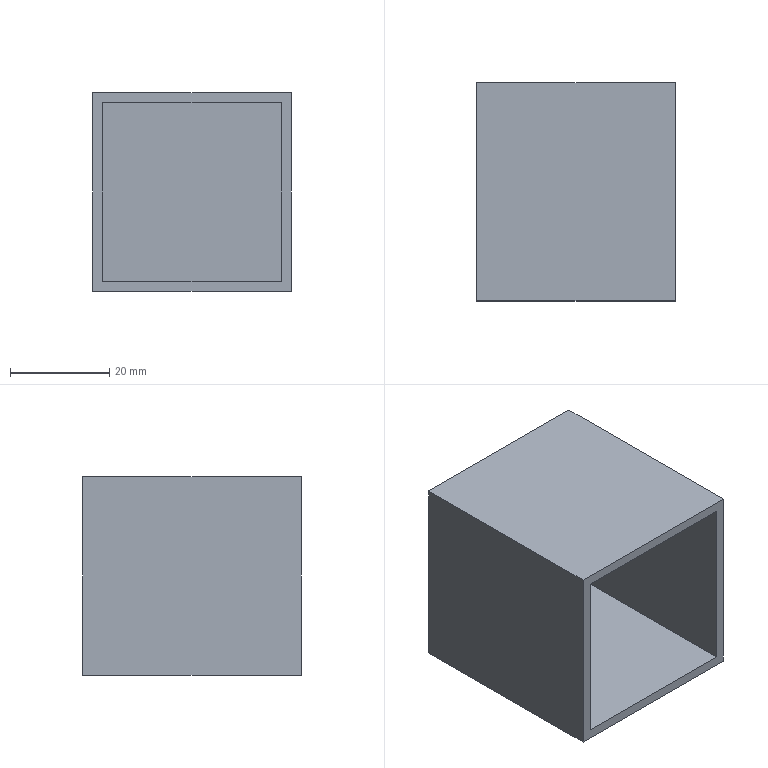Component | SolidWorks | Explosion-proofCasing-1 | 1 solid | 11 faces | box 40 x 44 x 40 mm | volume 15968 mm3 | plane 11 | material 45
build123d program:
from build123d import *

# Parameters (mm, degrees)
SKETCH1_W           = 40
SKETCH1_H           = 40
SKETCH1_W_2         = 36
SKETCH1_H_2         = 36
EXTRUDE_THIN1_DEPTH = 42
SKETCH2_W           = 40
SKETCH2_H           = 40
BOSS_EXTRUDE1_DEPTH = 2


with BuildPart() as part:
    # Sketch1 → Extrude-Thin1 (new body)
    with BuildSketch(Plane.XY):
        Rectangle(SKETCH1_W, SKETCH1_H)
        Rectangle(SKETCH1_W_2, SKETCH1_H_2, mode=Mode.SUBTRACT)
    extrude(amount=EXTRUDE_THIN1_DEPTH)

    # Sketch2 → Boss-Extrude1 (add)
    with BuildSketch(Plane(origin=(0, 0, 0), x_dir=(-1, 0, 0), z_dir=(0, 0, -1))):
        Rectangle(SKETCH2_W, SKETCH2_H)
    extrude(amount=BOSS_EXTRUDE1_DEPTH)


solid = part.part

# Placed as in the assembly
solid = solid.moved(Location((-371.359, -405.185, 1062), (90, 0, 0)))
STEP:
#1=COLOUR_RGB('',0.7922,0.8196,0.9333);
#2=FILL_AREA_STYLE_COLOUR('',#1);
#3=FILL_AREA_STYLE('',(#2));
#4=SURFACE_STYLE_FILL_AREA(#3);
#5=SURFACE_SIDE_STYLE('',(#4));
#6=SURFACE_STYLE_USAGE(.BOTH.,#5);
#7=PRESENTATION_STYLE_ASSIGNMENT((#6));
#8=CARTESIAN_POINT('',(-15.408,-17.606,42.598));
#9=VERTEX_POINT('',#8);
#10=CARTESIAN_POINT('',(-15.408,-17.606,41.024));
#11=VERTEX_POINT('',#10);
#12=CARTESIAN_POINT('',(-15.408,-17.606,41.024));
#13=DIRECTION('',(-0.,0.,-1.));
#14=VECTOR('',#13,39.37);
#15=LINE('',#12,#14);
#16=EDGE_CURVE('',#9,#11,#15,.T.);
#17=ORIENTED_EDGE('',*,*,#16,.T.);
#18=CARTESIAN_POINT('',(-13.833,-17.606,41.024));
#19=VERTEX_POINT('',#18);
#20=CARTESIAN_POINT('',(-13.833,-17.606,41.024));
#21=DIRECTION('',(1.,0.,0.));
#22=VECTOR('',#21,39.37);
#23=LINE('',#20,#22);
#24=EDGE_CURVE('',#11,#19,#23,.T.);
#25=ORIENTED_EDGE('',*,*,#24,.T.);
#26=CARTESIAN_POINT('',(-13.833,-17.606,42.598));
#27=VERTEX_POINT('',#26);
#28=CARTESIAN_POINT('',(-13.833,-17.606,41.024));
#29=DIRECTION('',(0.,0.,1.));
#30=VECTOR('',#29,39.37);
#31=LINE('',#28,#30);
#32=EDGE_CURVE('',#19,#27,#31,.T.);
#33=ORIENTED_EDGE('',*,*,#32,.T.);
#34=CARTESIAN_POINT('',(-13.833,-17.606,42.598));
#35=DIRECTION('',(-1.,0.,-0.));
#36=VECTOR('',#35,39.37);
#37=LINE('',#34,#36);
#38=EDGE_CURVE('',#27,#9,#37,.T.);
#39=ORIENTED_EDGE('',*,*,#38,.T.);
#40=EDGE_LOOP('',(#17,#25,#33,#39));
#41=FACE_OUTER_BOUND('',#40,.T.);
#42=CARTESIAN_POINT('',(-15.329,-17.606,41.102));
#43=VERTEX_POINT('',#42);
#44=CARTESIAN_POINT('',(-13.912,-17.606,41.102));
#45=VERTEX_POINT('',#44);
#46=CARTESIAN_POINT('',(-13.833,-17.606,41.102));
#47=DIRECTION('',(1.,0.,0.));
#48=VECTOR('',#47,39.37);
#49=LINE('',#46,#48);
#50=EDGE_CURVE('',#43,#45,#49,.T.);
#51=ORIENTED_EDGE('',*,*,#50,.F.);
#52=CARTESIAN_POINT('',(-15.329,-17.606,42.52));
#53=VERTEX_POINT('',#52);
#54=CARTESIAN_POINT('',(-15.329,-17.606,41.024));
#55=DIRECTION('',(-0.,0.,-1.));
#56=VECTOR('',#55,39.37);
#57=LINE('',#54,#56);
#58=EDGE_CURVE('',#53,#43,#57,.T.);
#59=ORIENTED_EDGE('',*,*,#58,.F.);
#60=CARTESIAN_POINT('',(-13.912,-17.606,42.52));
#61=VERTEX_POINT('',#60);
#62=CARTESIAN_POINT('',(-13.833,-17.606,42.52));
#63=DIRECTION('',(-1.,0.,-0.));
#64=VECTOR('',#63,39.37);
#65=LINE('',#62,#64);
#66=EDGE_CURVE('',#61,#53,#65,.T.);
#67=ORIENTED_EDGE('',*,*,#66,.F.);
#68=CARTESIAN_POINT('',(-13.912,-17.606,41.024));
#69=DIRECTION('',(0.,0.,1.));
#70=VECTOR('',#69,39.37);
#71=LINE('',#68,#70);
#72=EDGE_CURVE('',#45,#61,#71,.T.);
#73=ORIENTED_EDGE('',*,*,#72,.F.);
#74=EDGE_LOOP('',(#51,#59,#67,#73));
#75=FACE_BOUND('',#74,.T.);
#76=CARTESIAN_POINT('',(-14.62,-17.606,41.811));
#77=DIRECTION('',(0.,-1.,0.));
#78=DIRECTION('',(1.,0.,0.));
#79=AXIS2_PLACEMENT_3D('',#76,#77,#78);
#80=PLANE('',#79);
#81=ADVANCED_FACE('',(#41,#75),#80,.T.);
#82=CARTESIAN_POINT('',(-15.408,-15.873,42.598));
#83=VERTEX_POINT('',#82);
#84=CARTESIAN_POINT('',(-15.408,-17.606,42.598));
#85=DIRECTION('',(0.,1.,0.));
#86=VECTOR('',#85,39.37);
#87=LINE('',#84,#86);
#88=EDGE_CURVE('',#9,#83,#87,.T.);
#89=ORIENTED_EDGE('',*,*,#88,.T.);
#90=CARTESIAN_POINT('',(-15.408,-15.873,41.024));
#91=VERTEX_POINT('',#90);
#92=CARTESIAN_POINT('',(-15.408,-15.873,41.024));
#93=DIRECTION('',(0.,0.,1.));
#94=VECTOR('',#93,39.37);
#95=LINE('',#92,#94);
#96=EDGE_CURVE('',#91,#83,#95,.T.);
#97=ORIENTED_EDGE('',*,*,#96,.F.);
#98=CARTESIAN_POINT('',(-15.408,-17.606,41.024));
#99=DIRECTION('',(0.,1.,0.));
#100=VECTOR('',#99,39.37);
#101=LINE('',#98,#100);
#102=EDGE_CURVE('',#11,#91,#101,.T.);
#103=ORIENTED_EDGE('',*,*,#102,.F.);
#104=ORIENTED_EDGE('',*,*,#16,.F.);
#105=EDGE_LOOP('',(#89,#97,#103,#104));
#106=FACE_OUTER_BOUND('',#105,.T.);
#107=CARTESIAN_POINT('',(-15.408,-17.606,41.024));
#108=DIRECTION('',(1.,0.,-0.));
#109=DIRECTION('',(0.,0.,1.));
#110=AXIS2_PLACEMENT_3D('',#107,#108,#109);
#111=PLANE('',#110);
#112=ADVANCED_FACE('',(#106),#111,.F.);
#113=ORIENTED_EDGE('',*,*,#102,.T.);
#114=CARTESIAN_POINT('',(-13.833,-15.873,41.024));
#115=VERTEX_POINT('',#114);
#116=CARTESIAN_POINT('',(-13.833,-15.873,41.024));
#117=DIRECTION('',(-1.,0.,-0.));
#118=VECTOR('',#117,39.37);
#119=LINE('',#116,#118);
#120=EDGE_CURVE('',#115,#91,#119,.T.);
#121=ORIENTED_EDGE('',*,*,#120,.F.);
#122=CARTESIAN_POINT('',(-13.833,-17.606,41.024));
#123=DIRECTION('',(0.,1.,0.));
#124=VECTOR('',#123,39.37);
#125=LINE('',#122,#124);
#126=EDGE_CURVE('',#19,#115,#125,.T.);
#127=ORIENTED_EDGE('',*,*,#126,.F.);
#128=ORIENTED_EDGE('',*,*,#24,.F.);
#129=EDGE_LOOP('',(#113,#121,#127,#128));
#130=FACE_OUTER_BOUND('',#129,.T.);
#131=CARTESIAN_POINT('',(-13.833,-17.606,41.024));
#132=DIRECTION('',(-0.,0.,1.));
#133=DIRECTION('',(-1.,0.,-0.));
#134=AXIS2_PLACEMENT_3D('',#131,#132,#133);
#135=PLANE('',#134);
#136=ADVANCED_FACE('',(#130),#135,.F.);
#137=ORIENTED_EDGE('',*,*,#126,.T.);
#138=CARTESIAN_POINT('',(-13.833,-15.873,42.598));
#139=VERTEX_POINT('',#138);
#140=CARTESIAN_POINT('',(-13.833,-15.873,42.598));
#141=DIRECTION('',(0.,0.,-1.));
#142=VECTOR('',#141,39.37);
#143=LINE('',#140,#142);
#144=EDGE_CURVE('',#139,#115,#143,.T.);
#145=ORIENTED_EDGE('',*,*,#144,.F.);
#146=CARTESIAN_POINT('',(-13.833,-17.606,42.598));
#147=DIRECTION('',(0.,1.,0.));
#148=VECTOR('',#147,39.37);
#149=LINE('',#146,#148);
#150=EDGE_CURVE('',#27,#139,#149,.T.);
#151=ORIENTED_EDGE('',*,*,#150,.F.);
#152=ORIENTED_EDGE('',*,*,#32,.F.);
#153=EDGE_LOOP('',(#137,#145,#151,#152));
#154=FACE_OUTER_BOUND('',#153,.T.);
#155=CARTESIAN_POINT('',(-13.833,-17.606,41.024));
#156=DIRECTION('',(-1.,0.,0.));
#157=DIRECTION('',(0.,-1.,0.));
#158=AXIS2_PLACEMENT_3D('',#155,#156,#157);
#159=PLANE('',#158);
#160=ADVANCED_FACE('',(#154),#159,.F.);
#161=ORIENTED_EDGE('',*,*,#150,.T.);
#162=CARTESIAN_POINT('',(-15.408,-15.873,42.598));
#163=DIRECTION('',(1.,0.,0.));
#164=VECTOR('',#163,39.37);
#165=LINE('',#162,#164);
#166=EDGE_CURVE('',#83,#139,#165,.T.);
#167=ORIENTED_EDGE('',*,*,#166,.F.);
#168=ORIENTED_EDGE('',*,*,#88,.F.);
#169=ORIENTED_EDGE('',*,*,#38,.F.);
#170=EDGE_LOOP('',(#161,#167,#168,#169));
#171=FACE_OUTER_BOUND('',#170,.T.);
#172=CARTESIAN_POINT('',(-13.833,-17.606,42.598));
#173=DIRECTION('',(0.,0.,-1.));
#174=DIRECTION('',(1.,0.,0.));
#175=AXIS2_PLACEMENT_3D('',#172,#173,#174);
#176=PLANE('',#175);
#177=ADVANCED_FACE('',(#171),#176,.F.);
#178=CARTESIAN_POINT('',(-15.329,-15.952,42.52));
#179=VERTEX_POINT('',#178);
#180=CARTESIAN_POINT('',(-15.329,-15.952,41.102));
#181=VERTEX_POINT('',#180);
#182=CARTESIAN_POINT('',(-15.329,-15.952,41.024));
#183=DIRECTION('',(-0.,0.,-1.));
#184=VECTOR('',#183,39.37);
#185=LINE('',#182,#184);
#186=EDGE_CURVE('',#179,#181,#185,.T.);
#187=ORIENTED_EDGE('',*,*,#186,.F.);
#188=CARTESIAN_POINT('',(-15.329,-17.606,42.52));
#189=DIRECTION('',(0.,1.,0.));
#190=VECTOR('',#189,39.37);
#191=LINE('',#188,#190);
#192=EDGE_CURVE('',#53,#179,#191,.T.);
#193=ORIENTED_EDGE('',*,*,#192,.F.);
#194=ORIENTED_EDGE('',*,*,#58,.T.);
#195=CARTESIAN_POINT('',(-15.329,-17.606,41.102));
#196=DIRECTION('',(0.,1.,0.));
#197=VECTOR('',#196,39.37);
#198=LINE('',#195,#197);
#199=EDGE_CURVE('',#43,#181,#198,.T.);
#200=ORIENTED_EDGE('',*,*,#199,.T.);
#201=EDGE_LOOP('',(#187,#193,#194,#200));
#202=FACE_OUTER_BOUND('',#201,.T.);
#203=CARTESIAN_POINT('',(-15.329,-17.606,41.024));
#204=DIRECTION('',(1.,0.,-0.));
#205=DIRECTION('',(0.,0.,1.));
#206=AXIS2_PLACEMENT_3D('',#203,#204,#205);
#207=PLANE('',#206);
#208=ADVANCED_FACE('',(#202),#207,.T.);
#209=CARTESIAN_POINT('',(-13.912,-15.952,41.102));
#210=VERTEX_POINT('',#209);
#211=CARTESIAN_POINT('',(-13.833,-15.952,41.102));
#212=DIRECTION('',(1.,0.,0.));
#213=VECTOR('',#212,39.37);
#214=LINE('',#211,#213);
#215=EDGE_CURVE('',#181,#210,#214,.T.);
#216=ORIENTED_EDGE('',*,*,#215,.F.);
#217=ORIENTED_EDGE('',*,*,#199,.F.);
#218=ORIENTED_EDGE('',*,*,#50,.T.);
#219=CARTESIAN_POINT('',(-13.912,-17.606,41.102));
#220=DIRECTION('',(0.,1.,0.));
#221=VECTOR('',#220,39.37);
#222=LINE('',#219,#221);
#223=EDGE_CURVE('',#45,#210,#222,.T.);
#224=ORIENTED_EDGE('',*,*,#223,.T.);
#225=EDGE_LOOP('',(#216,#217,#218,#224));
#226=FACE_OUTER_BOUND('',#225,.T.);
#227=CARTESIAN_POINT('',(-13.833,-17.606,41.102));
#228=DIRECTION('',(-0.,0.,1.));
#229=DIRECTION('',(-1.,0.,-0.));
#230=AXIS2_PLACEMENT_3D('',#227,#228,#229);
#231=PLANE('',#230);
#232=ADVANCED_FACE('',(#226),#231,.T.);
#233=CARTESIAN_POINT('',(-13.912,-15.952,42.52));
#234=VERTEX_POINT('',#233);
#235=CARTESIAN_POINT('',(-13.912,-15.952,41.024));
#236=DIRECTION('',(0.,0.,1.));
#237=VECTOR('',#236,39.37);
#238=LINE('',#235,#237);
#239=EDGE_CURVE('',#210,#234,#238,.T.);
#240=ORIENTED_EDGE('',*,*,#239,.F.);
#241=ORIENTED_EDGE('',*,*,#223,.F.);
#242=ORIENTED_EDGE('',*,*,#72,.T.);
#243=CARTESIAN_POINT('',(-13.912,-17.606,42.52));
#244=DIRECTION('',(0.,1.,0.));
#245=VECTOR('',#244,39.37);
#246=LINE('',#243,#245);
#247=EDGE_CURVE('',#61,#234,#246,.T.);
#248=ORIENTED_EDGE('',*,*,#247,.T.);
#249=EDGE_LOOP('',(#240,#241,#242,#248));
#250=FACE_OUTER_BOUND('',#249,.T.);
#251=CARTESIAN_POINT('',(-13.912,-17.606,41.024));
#252=DIRECTION('',(-1.,0.,0.));
#253=DIRECTION('',(0.,-1.,0.));
#254=AXIS2_PLACEMENT_3D('',#251,#252,#253);
#255=PLANE('',#254);
#256=ADVANCED_FACE('',(#250),#255,.T.);
#257=CARTESIAN_POINT('',(-13.833,-15.952,42.52));
#258=DIRECTION('',(-1.,0.,-0.));
#259=VECTOR('',#258,39.37);
#260=LINE('',#257,#259);
#261=EDGE_CURVE('',#234,#179,#260,.T.);
#262=ORIENTED_EDGE('',*,*,#261,.F.);
#263=ORIENTED_EDGE('',*,*,#247,.F.);
#264=ORIENTED_EDGE('',*,*,#66,.T.);
#265=ORIENTED_EDGE('',*,*,#192,.T.);
#266=EDGE_LOOP('',(#262,#263,#264,#265));
#267=FACE_OUTER_BOUND('',#266,.T.);
#268=CARTESIAN_POINT('',(-13.833,-17.606,42.52));
#269=DIRECTION('',(0.,0.,-1.));
#270=DIRECTION('',(1.,0.,0.));
#271=AXIS2_PLACEMENT_3D('',#268,#269,#270);
#272=PLANE('',#271);
#273=ADVANCED_FACE('',(#267),#272,.T.);
#274=ORIENTED_EDGE('',*,*,#261,.T.);
#275=ORIENTED_EDGE('',*,*,#186,.T.);
#276=ORIENTED_EDGE('',*,*,#215,.T.);
#277=ORIENTED_EDGE('',*,*,#239,.T.);
#278=EDGE_LOOP('',(#274,#275,#276,#277));
#279=FACE_OUTER_BOUND('',#278,.T.);
#280=CARTESIAN_POINT('',(-14.62,-15.952,41.811));
#281=DIRECTION('',(0.,1.,0.));
#282=DIRECTION('',(-1.,0.,0.));
#283=AXIS2_PLACEMENT_3D('',#280,#281,#282);
#284=PLANE('',#283);
#285=ADVANCED_FACE('',(#279),#284,.F.);
#286=ORIENTED_EDGE('',*,*,#120,.T.);
#287=ORIENTED_EDGE('',*,*,#96,.T.);
#288=ORIENTED_EDGE('',*,*,#166,.T.);
#289=ORIENTED_EDGE('',*,*,#144,.T.);
#290=EDGE_LOOP('',(#286,#287,#288,#289));
#291=FACE_OUTER_BOUND('',#290,.T.);
#292=CARTESIAN_POINT('',(-14.62,-15.873,41.811));
#293=DIRECTION('',(0.,1.,0.));
#294=DIRECTION('',(-1.,0.,0.));
#295=AXIS2_PLACEMENT_3D('',#292,#293,#294);
#296=PLANE('',#295);
#297=ADVANCED_FACE('',(#291),#296,.T.);
#298=CLOSED_SHELL('',(#81,#112,#136,#160,#177,#208,#232,#256,#273,#285,#297));
#299=MANIFOLD_SOLID_BREP('',#298);
#300=STYLED_ITEM('',(#7),#299);
#301=PRESENTATION_LAYER_ASSIGNMENT('','',(#300));
#302=CARTESIAN_POINT('',(0.,0.,0.));
#303=DIRECTION('',(0.,0.,1.));
#304=DIRECTION('',(1.,0.,0.));
#305=AXIS2_PLACEMENT_3D('',#302,#303,#304);
#306=(LENGTH_UNIT()NAMED_UNIT(*)SI_UNIT($,.METRE.));
#307=LENGTH_MEASURE_WITH_UNIT(LENGTH_MEASURE(0.0254),#306);
#308=DIMENSIONAL_EXPONENTS(1.,0.,0.,0.,0.,0.,0.);
#309=(CONVERSION_BASED_UNIT('',#307)LENGTH_UNIT()NAMED_UNIT(#308));
#310=UNCERTAINTY_MEASURE_WITH_UNIT(LENGTH_MEASURE(0.00001),#309,'','');
#311=(NAMED_UNIT(*)PLANE_ANGLE_UNIT()SI_UNIT($,.RADIAN.));
#312=(NAMED_UNIT(*)SI_UNIT($,.STERADIAN.)SOLID_ANGLE_UNIT());
#313=(GEOMETRIC_REPRESENTATION_CONTEXT(3)GLOBAL_UNCERTAINTY_ASSIGNED_CONTEXT((#310))GLOBAL_UNIT_ASSIGNED_CONTEXT((#309,#311,#312))REPRESENTATION_CONTEXT('',''));
#314=ADVANCED_BREP_SHAPE_REPRESENTATION('',(#299,#305),#313);
#315=(LENGTH_UNIT()NAMED_UNIT(*)SI_UNIT($,.METRE.));
#316=LENGTH_MEASURE_WITH_UNIT(LENGTH_MEASURE(0.0254),#315);
#317=DIMENSIONAL_EXPONENTS(1.,0.,0.,0.,0.,0.,0.);
#318=(CONVERSION_BASED_UNIT('',#316)LENGTH_UNIT()NAMED_UNIT(#317));
#319=UNCERTAINTY_MEASURE_WITH_UNIT(LENGTH_MEASURE(0.00001),#318,'','');
#320=(NAMED_UNIT(*)PLANE_ANGLE_UNIT()SI_UNIT($,.RADIAN.));
#321=(NAMED_UNIT(*)SI_UNIT($,.STERADIAN.)SOLID_ANGLE_UNIT());
#322=(GEOMETRIC_REPRESENTATION_CONTEXT(3)GLOBAL_UNCERTAINTY_ASSIGNED_CONTEXT((#319))GLOBAL_UNIT_ASSIGNED_CONTEXT((#318,#320,#321))REPRESENTATION_CONTEXT('',''));
#323=MECHANICAL_DESIGN_GEOMETRIC_PRESENTATION_REPRESENTATION('',(#300),#322);